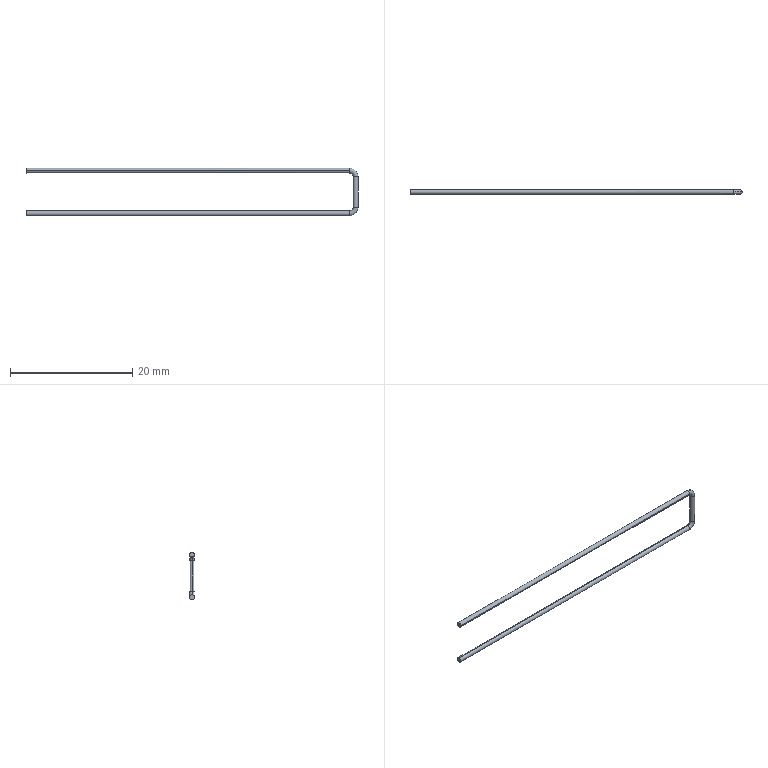Component | SolidWorks | TailWing-1 | 1 solid | 12 faces | box 54.4 x 0.8 x 7.8 mm | volume 57 mm3 | cylinder 6 | torus 4 | plane 2 | commonest cylinder face diameters 0.8 x6
STEP:
#1=CARTESIAN_POINT('',(2.772,0.1969,0.1378));
#2=VERTEX_POINT('',#1);
#3=CARTESIAN_POINT('',(2.74,0.1969,0.1378));
#4=VERTEX_POINT('',#3);
#5=CARTESIAN_POINT('',(2.756,0.1969,0.1378));
#6=DIRECTION('',(0.,0.,-1.));
#7=DIRECTION('',(-1.,0.,0.));
#8=AXIS2_PLACEMENT_3D('',#5,#6,#7);
#9=CIRCLE('',#8,0.01575);
#10=EDGE_CURVE('',#2,#4,#9,.T.);
#11=ORIENTED_EDGE('',*,*,#10,.F.);
#12=CARTESIAN_POINT('',(2.717,0.1969,0.1929));
#13=VERTEX_POINT('',#12);
#14=CARTESIAN_POINT('',(2.717,0.1969,0.1378));
#15=DIRECTION('',(-0.,-1.,0.));
#16=DIRECTION('',(1.,0.,0.));
#17=AXIS2_PLACEMENT_3D('',#14,#15,#16);
#18=CIRCLE('',#17,0.05512);
#19=EDGE_CURVE('',#2,#13,#18,.T.);
#20=ORIENTED_EDGE('',*,*,#19,.T.);
#21=CARTESIAN_POINT('',(2.717,0.1811,0.1772));
#22=VERTEX_POINT('',#21);
#23=CARTESIAN_POINT('',(2.717,0.1969,0.1772));
#24=DIRECTION('',(1.,0.,0.));
#25=DIRECTION('',(0.,0.,-1.));
#26=AXIS2_PLACEMENT_3D('',#23,#24,#25);
#27=CIRCLE('',#26,0.01575);
#28=EDGE_CURVE('',#13,#22,#27,.T.);
#29=ORIENTED_EDGE('',*,*,#28,.T.);
#30=CARTESIAN_POINT('',(2.717,0.1969,0.1614));
#31=VERTEX_POINT('',#30);
#32=CARTESIAN_POINT('',(2.717,0.1969,0.1772));
#33=DIRECTION('',(1.,0.,0.));
#34=DIRECTION('',(0.,0.,-1.));
#35=AXIS2_PLACEMENT_3D('',#32,#33,#34);
#36=CIRCLE('',#35,0.01575);
#37=EDGE_CURVE('',#22,#31,#36,.T.);
#38=ORIENTED_EDGE('',*,*,#37,.T.);
#39=CARTESIAN_POINT('',(2.717,0.1969,0.1378));
#40=DIRECTION('',(-0.,-1.,0.));
#41=DIRECTION('',(1.,0.,0.));
#42=AXIS2_PLACEMENT_3D('',#39,#40,#41);
#43=CIRCLE('',#42,0.02362);
#44=EDGE_CURVE('',#4,#31,#43,.T.);
#45=ORIENTED_EDGE('',*,*,#44,.F.);
#46=EDGE_LOOP('',(#11,#20,#29,#38,#45));
#47=FACE_OUTER_BOUND('',#46,.T.);
#48=CARTESIAN_POINT('',(2.717,0.1969,0.1378));
#49=DIRECTION('',(-0.,-1.,0.));
#50=DIRECTION('',(1.,-0.,0.));
#51=AXIS2_PLACEMENT_3D('',#48,#49,#50);
#52=TOROIDAL_SURFACE('',#51,0.03937,0.01575);
#53=ADVANCED_FACE('',(#47),#52,.T.);
#54=CARTESIAN_POINT('',(2.717,0.1969,-0.1142));
#55=VERTEX_POINT('',#54);
#56=CARTESIAN_POINT('',(2.717,0.1969,-0.08268));
#57=VERTEX_POINT('',#56);
#58=CARTESIAN_POINT('',(2.717,0.1969,-0.09843));
#59=DIRECTION('',(-1.,0.,0.));
#60=DIRECTION('',(0.,0.,1.));
#61=AXIS2_PLACEMENT_3D('',#58,#59,#60);
#62=CIRCLE('',#61,0.01575);
#63=EDGE_CURVE('',#55,#57,#62,.T.);
#64=ORIENTED_EDGE('',*,*,#63,.F.);
#65=CARTESIAN_POINT('',(2.772,0.1969,-0.05906));
#66=VERTEX_POINT('',#65);
#67=CARTESIAN_POINT('',(2.717,0.1969,-0.05906));
#68=DIRECTION('',(-0.,-1.,0.));
#69=DIRECTION('',(1.,0.,0.));
#70=AXIS2_PLACEMENT_3D('',#67,#68,#69);
#71=CIRCLE('',#70,0.05512);
#72=EDGE_CURVE('',#55,#66,#71,.T.);
#73=ORIENTED_EDGE('',*,*,#72,.T.);
#74=CARTESIAN_POINT('',(2.74,0.1969,-0.05906));
#75=VERTEX_POINT('',#74);
#76=CARTESIAN_POINT('',(2.756,0.1969,-0.05906));
#77=DIRECTION('',(0.,0.,-1.));
#78=DIRECTION('',(-1.,0.,0.));
#79=AXIS2_PLACEMENT_3D('',#76,#77,#78);
#80=CIRCLE('',#79,0.01575);
#81=EDGE_CURVE('',#66,#75,#80,.T.);
#82=ORIENTED_EDGE('',*,*,#81,.T.);
#83=CARTESIAN_POINT('',(2.717,0.1969,-0.05906));
#84=DIRECTION('',(-0.,-1.,0.));
#85=DIRECTION('',(1.,0.,0.));
#86=AXIS2_PLACEMENT_3D('',#83,#84,#85);
#87=CIRCLE('',#86,0.02362);
#88=EDGE_CURVE('',#57,#75,#87,.T.);
#89=ORIENTED_EDGE('',*,*,#88,.F.);
#90=EDGE_LOOP('',(#64,#73,#82,#89));
#91=FACE_OUTER_BOUND('',#90,.T.);
#92=CARTESIAN_POINT('',(2.717,0.1969,-0.05906));
#93=DIRECTION('',(-0.,-1.,0.));
#94=DIRECTION('',(1.,-0.,0.));
#95=AXIS2_PLACEMENT_3D('',#92,#93,#94);
#96=TOROIDAL_SURFACE('',#95,0.03937,0.01575);
#97=ADVANCED_FACE('',(#91),#96,.T.);
#98=CARTESIAN_POINT('',(2.717,0.2126,0.1772));
#99=VERTEX_POINT('',#98);
#100=CARTESIAN_POINT('',(2.717,0.1969,0.1772));
#101=DIRECTION('',(1.,0.,0.));
#102=DIRECTION('',(0.,0.,-1.));
#103=AXIS2_PLACEMENT_3D('',#100,#101,#102);
#104=CIRCLE('',#103,0.01575);
#105=EDGE_CURVE('',#99,#13,#104,.T.);
#106=ORIENTED_EDGE('',*,*,#105,.F.);
#107=CARTESIAN_POINT('',(0.6299,0.2126,0.1772));
#108=VERTEX_POINT('',#107);
#109=CARTESIAN_POINT('',(2.717,0.2126,0.1772));
#110=DIRECTION('',(-1.,0.,0.));
#111=VECTOR('',#110,39.37);
#112=LINE('',#109,#111);
#113=EDGE_CURVE('',#99,#108,#112,.T.);
#114=ORIENTED_EDGE('',*,*,#113,.T.);
#115=CARTESIAN_POINT('',(0.6299,0.1811,0.1772));
#116=VERTEX_POINT('',#115);
#117=CARTESIAN_POINT('',(0.6299,0.1969,0.1772));
#118=DIRECTION('',(-1.,0.,0.));
#119=DIRECTION('',(0.,0.,1.));
#120=AXIS2_PLACEMENT_3D('',#117,#118,#119);
#121=CIRCLE('',#120,0.01575);
#122=EDGE_CURVE('',#116,#108,#121,.T.);
#123=ORIENTED_EDGE('',*,*,#122,.F.);
#124=CARTESIAN_POINT('',(2.717,0.1811,0.1772));
#125=DIRECTION('',(-1.,0.,0.));
#126=VECTOR('',#125,39.37);
#127=LINE('',#124,#126);
#128=EDGE_CURVE('',#22,#116,#127,.T.);
#129=ORIENTED_EDGE('',*,*,#128,.F.);
#130=ORIENTED_EDGE('',*,*,#28,.F.);
#131=EDGE_LOOP('',(#106,#114,#123,#129,#130));
#132=FACE_OUTER_BOUND('',#131,.T.);
#133=CARTESIAN_POINT('',(2.717,0.1969,0.1772));
#134=DIRECTION('',(-1.,0.,0.));
#135=DIRECTION('',(0.,-1.,0.));
#136=AXIS2_PLACEMENT_3D('',#133,#134,#135);
#137=CYLINDRICAL_SURFACE('',#136,0.01575);
#138=ADVANCED_FACE('',(#132),#137,.T.);
#139=CARTESIAN_POINT('',(2.756,0.1969,-0.05906));
#140=DIRECTION('',(0.,0.,-1.));
#141=DIRECTION('',(-1.,0.,0.));
#142=AXIS2_PLACEMENT_3D('',#139,#140,#141);
#143=CIRCLE('',#142,0.01575);
#144=EDGE_CURVE('',#75,#66,#143,.T.);
#145=ORIENTED_EDGE('',*,*,#144,.F.);
#146=CARTESIAN_POINT('',(2.74,0.1969,-0.05906));
#147=DIRECTION('',(0.,0.,1.));
#148=VECTOR('',#147,39.37);
#149=LINE('',#146,#148);
#150=EDGE_CURVE('',#75,#4,#149,.T.);
#151=ORIENTED_EDGE('',*,*,#150,.T.);
#152=CARTESIAN_POINT('',(2.756,0.1969,0.1378));
#153=DIRECTION('',(0.,0.,-1.));
#154=DIRECTION('',(-1.,0.,0.));
#155=AXIS2_PLACEMENT_3D('',#152,#153,#154);
#156=CIRCLE('',#155,0.01575);
#157=EDGE_CURVE('',#4,#2,#156,.T.);
#158=ORIENTED_EDGE('',*,*,#157,.T.);
#159=CARTESIAN_POINT('',(2.772,0.1969,-0.05906));
#160=DIRECTION('',(0.,0.,1.));
#161=VECTOR('',#160,39.37);
#162=LINE('',#159,#161);
#163=EDGE_CURVE('',#66,#2,#162,.T.);
#164=ORIENTED_EDGE('',*,*,#163,.F.);
#165=EDGE_LOOP('',(#145,#151,#158,#164));
#166=FACE_OUTER_BOUND('',#165,.T.);
#167=CARTESIAN_POINT('',(2.756,0.1969,-0.05906));
#168=DIRECTION('',(0.,0.,1.));
#169=DIRECTION('',(1.,0.,0.));
#170=AXIS2_PLACEMENT_3D('',#167,#168,#169);
#171=CYLINDRICAL_SURFACE('',#170,0.01575);
#172=ADVANCED_FACE('',(#166),#171,.T.);
#173=CARTESIAN_POINT('',(2.717,0.1969,-0.09843));
#174=DIRECTION('',(-1.,0.,0.));
#175=DIRECTION('',(0.,0.,1.));
#176=AXIS2_PLACEMENT_3D('',#173,#174,#175);
#177=CIRCLE('',#176,0.01575);
#178=EDGE_CURVE('',#57,#55,#177,.T.);
#179=ORIENTED_EDGE('',*,*,#178,.T.);
#180=CARTESIAN_POINT('',(0.6299,0.1969,-0.1142));
#181=VERTEX_POINT('',#180);
#182=CARTESIAN_POINT('',(2.598,0.1969,-0.1142));
#183=DIRECTION('',(-1.,0.,0.));
#184=VECTOR('',#183,39.37);
#185=LINE('',#182,#184);
#186=EDGE_CURVE('',#55,#181,#185,.T.);
#187=ORIENTED_EDGE('',*,*,#186,.T.);
#188=CARTESIAN_POINT('',(0.6299,0.1969,-0.08268));
#189=VERTEX_POINT('',#188);
#190=CARTESIAN_POINT('',(0.6299,0.1969,-0.09843));
#191=DIRECTION('',(-1.,0.,0.));
#192=DIRECTION('',(0.,0.,1.));
#193=AXIS2_PLACEMENT_3D('',#190,#191,#192);
#194=CIRCLE('',#193,0.01575);
#195=EDGE_CURVE('',#189,#181,#194,.T.);
#196=ORIENTED_EDGE('',*,*,#195,.F.);
#197=CARTESIAN_POINT('',(2.598,0.1969,-0.08268));
#198=DIRECTION('',(-1.,0.,0.));
#199=VECTOR('',#198,39.37);
#200=LINE('',#197,#199);
#201=EDGE_CURVE('',#57,#189,#200,.T.);
#202=ORIENTED_EDGE('',*,*,#201,.F.);
#203=EDGE_LOOP('',(#179,#187,#196,#202));
#204=FACE_OUTER_BOUND('',#203,.T.);
#205=CARTESIAN_POINT('',(2.598,0.1969,-0.09843));
#206=DIRECTION('',(-1.,0.,0.));
#207=DIRECTION('',(0.,0.,1.));
#208=AXIS2_PLACEMENT_3D('',#205,#206,#207);
#209=CYLINDRICAL_SURFACE('',#208,0.01575);
#210=ADVANCED_FACE('',(#204),#209,.T.);
#211=ORIENTED_EDGE('',*,*,#186,.F.);
#212=ORIENTED_EDGE('',*,*,#63,.T.);
#213=ORIENTED_EDGE('',*,*,#201,.T.);
#214=CARTESIAN_POINT('',(0.6299,0.1969,-0.09843));
#215=DIRECTION('',(-1.,0.,0.));
#216=DIRECTION('',(0.,0.,1.));
#217=AXIS2_PLACEMENT_3D('',#214,#215,#216);
#218=CIRCLE('',#217,0.01575);
#219=EDGE_CURVE('',#181,#189,#218,.T.);
#220=ORIENTED_EDGE('',*,*,#219,.F.);
#221=EDGE_LOOP('',(#211,#212,#213,#220));
#222=FACE_OUTER_BOUND('',#221,.T.);
#223=CARTESIAN_POINT('',(2.598,0.1969,-0.09843));
#224=DIRECTION('',(-1.,0.,0.));
#225=DIRECTION('',(0.,0.,1.));
#226=AXIS2_PLACEMENT_3D('',#223,#224,#225);
#227=CYLINDRICAL_SURFACE('',#226,0.01575);
#228=ADVANCED_FACE('',(#222),#227,.T.);
#229=ORIENTED_EDGE('',*,*,#195,.T.);
#230=ORIENTED_EDGE('',*,*,#219,.T.);
#231=EDGE_LOOP('',(#229,#230));
#232=FACE_OUTER_BOUND('',#231,.T.);
#233=CARTESIAN_POINT('',(0.6299,0.1969,-0.09843));
#234=DIRECTION('',(-1.,0.,0.));
#235=DIRECTION('',(0.,0.,1.));
#236=AXIS2_PLACEMENT_3D('',#233,#234,#235);
#237=PLANE('',#236);
#238=ADVANCED_FACE('',(#232),#237,.T.);
#239=ORIENTED_EDGE('',*,*,#113,.F.);
#240=CARTESIAN_POINT('',(2.717,0.1969,0.1772));
#241=DIRECTION('',(1.,0.,0.));
#242=DIRECTION('',(0.,0.,-1.));
#243=AXIS2_PLACEMENT_3D('',#240,#241,#242);
#244=CIRCLE('',#243,0.01575);
#245=EDGE_CURVE('',#31,#99,#244,.T.);
#246=ORIENTED_EDGE('',*,*,#245,.F.);
#247=ORIENTED_EDGE('',*,*,#37,.F.);
#248=ORIENTED_EDGE('',*,*,#128,.T.);
#249=CARTESIAN_POINT('',(0.6299,0.1969,0.1772));
#250=DIRECTION('',(-1.,0.,0.));
#251=DIRECTION('',(0.,0.,1.));
#252=AXIS2_PLACEMENT_3D('',#249,#250,#251);
#253=CIRCLE('',#252,0.01575);
#254=EDGE_CURVE('',#108,#116,#253,.T.);
#255=ORIENTED_EDGE('',*,*,#254,.F.);
#256=EDGE_LOOP('',(#239,#246,#247,#248,#255));
#257=FACE_OUTER_BOUND('',#256,.T.);
#258=CARTESIAN_POINT('',(2.717,0.1969,0.1772));
#259=DIRECTION('',(-1.,0.,0.));
#260=DIRECTION('',(0.,-1.,0.));
#261=AXIS2_PLACEMENT_3D('',#258,#259,#260);
#262=CYLINDRICAL_SURFACE('',#261,0.01575);
#263=ADVANCED_FACE('',(#257),#262,.T.);
#264=ORIENTED_EDGE('',*,*,#19,.F.);
#265=ORIENTED_EDGE('',*,*,#157,.F.);
#266=ORIENTED_EDGE('',*,*,#44,.T.);
#267=ORIENTED_EDGE('',*,*,#245,.T.);
#268=ORIENTED_EDGE('',*,*,#105,.T.);
#269=EDGE_LOOP('',(#264,#265,#266,#267,#268));
#270=FACE_OUTER_BOUND('',#269,.T.);
#271=CARTESIAN_POINT('',(2.717,0.1969,0.1378));
#272=DIRECTION('',(-0.,-1.,0.));
#273=DIRECTION('',(1.,-0.,0.));
#274=AXIS2_PLACEMENT_3D('',#271,#272,#273);
#275=TOROIDAL_SURFACE('',#274,0.03937,0.01575);
#276=ADVANCED_FACE('',(#270),#275,.T.);
#277=ORIENTED_EDGE('',*,*,#150,.F.);
#278=ORIENTED_EDGE('',*,*,#81,.F.);
#279=ORIENTED_EDGE('',*,*,#163,.T.);
#280=ORIENTED_EDGE('',*,*,#10,.T.);
#281=EDGE_LOOP('',(#277,#278,#279,#280));
#282=FACE_OUTER_BOUND('',#281,.T.);
#283=CARTESIAN_POINT('',(2.756,0.1969,-0.05906));
#284=DIRECTION('',(0.,0.,1.));
#285=DIRECTION('',(1.,0.,0.));
#286=AXIS2_PLACEMENT_3D('',#283,#284,#285);
#287=CYLINDRICAL_SURFACE('',#286,0.01575);
#288=ADVANCED_FACE('',(#282),#287,.T.);
#289=ORIENTED_EDGE('',*,*,#72,.F.);
#290=ORIENTED_EDGE('',*,*,#178,.F.);
#291=ORIENTED_EDGE('',*,*,#88,.T.);
#292=ORIENTED_EDGE('',*,*,#144,.T.);
#293=EDGE_LOOP('',(#289,#290,#291,#292));
#294=FACE_OUTER_BOUND('',#293,.T.);
#295=CARTESIAN_POINT('',(2.717,0.1969,-0.05906));
#296=DIRECTION('',(-0.,-1.,0.));
#297=DIRECTION('',(1.,-0.,0.));
#298=AXIS2_PLACEMENT_3D('',#295,#296,#297);
#299=TOROIDAL_SURFACE('',#298,0.03937,0.01575);
#300=ADVANCED_FACE('',(#294),#299,.T.);
#301=ORIENTED_EDGE('',*,*,#122,.T.);
#302=ORIENTED_EDGE('',*,*,#254,.T.);
#303=EDGE_LOOP('',(#301,#302));
#304=FACE_OUTER_BOUND('',#303,.T.);
#305=CARTESIAN_POINT('',(0.6299,0.1969,0.1772));
#306=DIRECTION('',(-1.,0.,0.));
#307=DIRECTION('',(0.,0.,1.));
#308=AXIS2_PLACEMENT_3D('',#305,#306,#307);
#309=PLANE('',#308);
#310=ADVANCED_FACE('',(#304),#309,.T.);
#311=CLOSED_SHELL('',(#53,#97,#138,#172,#210,#228,#238,#263,#276,#288,#300,#310));
#312=MANIFOLD_SOLID_BREP('',#311);
#313=CARTESIAN_POINT('',(0.,0.,0.));
#314=DIRECTION('',(0.,0.,1.));
#315=DIRECTION('',(1.,0.,0.));
#316=AXIS2_PLACEMENT_3D('',#313,#314,#315);
#317=(LENGTH_UNIT()NAMED_UNIT(*)SI_UNIT($,.METRE.));
#318=LENGTH_MEASURE_WITH_UNIT(LENGTH_MEASURE(0.0254),#317);
#319=DIMENSIONAL_EXPONENTS(1.,0.,0.,0.,0.,0.,0.);
#320=(CONVERSION_BASED_UNIT('',#318)LENGTH_UNIT()NAMED_UNIT(#319));
#321=UNCERTAINTY_MEASURE_WITH_UNIT(LENGTH_MEASURE(0.00001),#320,'','');
#322=(NAMED_UNIT(*)PLANE_ANGLE_UNIT()SI_UNIT($,.RADIAN.));
#323=(NAMED_UNIT(*)SI_UNIT($,.STERADIAN.)SOLID_ANGLE_UNIT());
#324=(GEOMETRIC_REPRESENTATION_CONTEXT(3)GLOBAL_UNCERTAINTY_ASSIGNED_CONTEXT((#321))GLOBAL_UNIT_ASSIGNED_CONTEXT((#320,#322,#323))REPRESENTATION_CONTEXT('',''));
#325=ADVANCED_BREP_SHAPE_REPRESENTATION('',(#312,#316),#324);
#326=COLOUR_RGB('',0.7922,0.8196,0.9333);
#327=FILL_AREA_STYLE_COLOUR('',#326);
#328=FILL_AREA_STYLE('',(#327));
#329=SURFACE_STYLE_FILL_AREA(#328);
#330=SURFACE_SIDE_STYLE('',(#329));
#331=SURFACE_STYLE_USAGE(.BOTH.,#330);
#332=PRESENTATION_STYLE_ASSIGNMENT((#331));
#333=STYLED_ITEM('',(#332),#312);
#334=(LENGTH_UNIT()NAMED_UNIT(*)SI_UNIT($,.METRE.));
#335=LENGTH_MEASURE_WITH_UNIT(LENGTH_MEASURE(0.0254),#334);
#336=DIMENSIONAL_EXPONENTS(1.,0.,0.,0.,0.,0.,0.);
#337=(CONVERSION_BASED_UNIT('',#335)LENGTH_UNIT()NAMED_UNIT(#336));
#338=UNCERTAINTY_MEASURE_WITH_UNIT(LENGTH_MEASURE(0.00001),#337,'','');
#339=(NAMED_UNIT(*)PLANE_ANGLE_UNIT()SI_UNIT($,.RADIAN.));
#340=(NAMED_UNIT(*)SI_UNIT($,.STERADIAN.)SOLID_ANGLE_UNIT());
#341=(GEOMETRIC_REPRESENTATION_CONTEXT(3)GLOBAL_UNCERTAINTY_ASSIGNED_CONTEXT((#338))GLOBAL_UNIT_ASSIGNED_CONTEXT((#337,#339,#340))REPRESENTATION_CONTEXT('',''));
#342=MECHANICAL_DESIGN_GEOMETRIC_PRESENTATION_REPRESENTATION('',(#333),#341);
#343=PRESENTATION_LAYER_ASSIGNMENT('','',(#333));